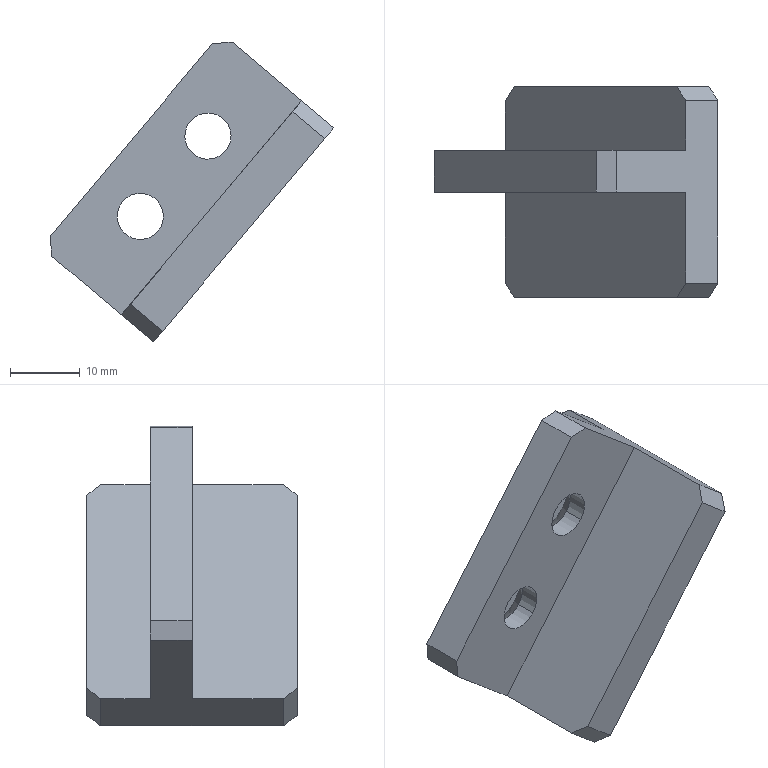Component | SolidWorks | 05CameraLensMountPlate-1 | 1 solid | 24 faces | box 40.54 x 30.1 x 42.84 mm | volume 10080 mm3 | plane 16 | cone 4 | cylinder 4 | commonest cylinder face diameters 6.6 x4 | material Aviation Aluminum-7075
build123d program:
from build123d import *

# Parameters (mm, degrees)
SKETCH1_W                                          = 40
SKETCH1_H                                          = 30.1
BOSS_EXTRUDE1_DEPTH                                = 6
SKETCH2_W                                          = 40
SKETCH2_H                                          = 6
BOSS_EXTRUDE2_DEPTH                                = 15
CHAMFER1_SIZE                                      = 2
HOLE_SIZE_ACCORDING_TO_TYPE_1_OF_HEXAG_D           = 6.6
HOLE_SIZE_ACCORDING_TO_TYPE_1_OF_HEXAG_DEPTH       = 15
HOLE_SIZE_ACCORDING_TO_TYPE_1_OF_HEXAG_CSINK_D     = 12.8
HOLE_SIZE_ACCORDING_TO_TYPE_1_OF_HEXAG_CSINK_ANGLE = 90
HOLE_SIZE_ACCORDING_TO_TYPE_1_OF_HEXAG_TIP         = 1.983


with BuildPart() as part:
    # Sketch1 → Boss-Extrude1 (new body)
    with BuildSketch(Plane.XY):
        Rectangle(SKETCH1_W, SKETCH1_H)
    extrude(amount=BOSS_EXTRUDE1_DEPTH)

    # Sketch2 → Boss-Extrude2 (add)
    with BuildSketch(Plane.XY.offset(6)):
        with Locations((0, -2.95)):
            Rectangle(SKETCH2_W, SKETCH2_H)
    extrude(amount=BOSS_EXTRUDE2_DEPTH)

    # Chamfer1
    chamfer1_edges = [part.edges().sort_by_distance(p)[0] for p in [
        (-20, -2.95, 21),
        (20, -2.95, 21),
        (-20, 15.05, 3),
        (20, 15.05, 3),
        (20, -15.05, 3),
        (-20, -15.05, 3),
    ]]
    chamfer(chamfer1_edges, length=CHAMFER1_SIZE)

    # Hole Size _According to_ Type 1 of Hexag
    with Locations(Plane(origin=(7.5, -5.95, 13), x_dir=(0, 0, -1), z_dir=(0, -1, 0))):
        with Locations((0, 0), (0, -15)):
            CounterSinkHole(HOLE_SIZE_ACCORDING_TO_TYPE_1_OF_HEXAG_D / 2, HOLE_SIZE_ACCORDING_TO_TYPE_1_OF_HEXAG_CSINK_D / 2, depth=HOLE_SIZE_ACCORDING_TO_TYPE_1_OF_HEXAG_DEPTH, counter_sink_angle=HOLE_SIZE_ACCORDING_TO_TYPE_1_OF_HEXAG_CSINK_ANGLE)
            with Locations((0, 0, -(HOLE_SIZE_ACCORDING_TO_TYPE_1_OF_HEXAG_DEPTH + HOLE_SIZE_ACCORDING_TO_TYPE_1_OF_HEXAG_TIP / 2))):  # 118° drill point
                Cone(0, HOLE_SIZE_ACCORDING_TO_TYPE_1_OF_HEXAG_D / 2, HOLE_SIZE_ACCORDING_TO_TYPE_1_OF_HEXAG_TIP, mode=Mode.SUBTRACT)


solid = part.part

# Placed as in the assembly
solid = solid.moved(Location((-338.792, 164.695, -100.519), (0, -49.905, -180)))
STEP:
#1=COLOUR_RGB('',0.7922,0.8196,0.9333);
#2=FILL_AREA_STYLE_COLOUR('',#1);
#3=FILL_AREA_STYLE('',(#2));
#4=SURFACE_STYLE_FILL_AREA(#3);
#5=SURFACE_SIDE_STYLE('',(#4));
#6=SURFACE_STYLE_USAGE(.BOTH.,#5);
#7=PRESENTATION_STYLE_ASSIGNMENT((#6));
#8=CARTESIAN_POINT('',(-14.019,6.596,-3.77));
#9=VERTEX_POINT('',#8);
#10=CARTESIAN_POINT('',(-13.821,6.596,-3.937));
#11=VERTEX_POINT('',#10);
#12=CARTESIAN_POINT('',(-13.92,6.596,-3.854));
#13=DIRECTION('',(-0.,1.,0.));
#14=DIRECTION('',(0.765,0.,-0.6441));
#15=AXIS2_PLACEMENT_3D('',#12,#13,#14);
#16=CIRCLE('',#15,0.1299);
#17=EDGE_CURVE('',#9,#11,#16,.T.);
#18=ORIENTED_EDGE('',*,*,#17,.F.);
#19=CARTESIAN_POINT('',(-14.113,6.718,-3.691));
#20=VERTEX_POINT('',#19);
#21=CARTESIAN_POINT('',(-14.113,6.718,-3.691));
#22=DIRECTION('',(-0.5409,0.7071,0.4554));
#23=VECTOR('',#22,39.37);
#24=LINE('',#21,#23);
#25=EDGE_CURVE('',#9,#20,#24,.T.);
#26=ORIENTED_EDGE('',*,*,#25,.T.);
#27=CARTESIAN_POINT('',(-13.727,6.718,-4.016));
#28=VERTEX_POINT('',#27);
#29=CARTESIAN_POINT('',(-13.92,6.718,-3.854));
#30=DIRECTION('',(-0.,1.,0.));
#31=DIRECTION('',(0.765,0.,-0.6441));
#32=AXIS2_PLACEMENT_3D('',#29,#30,#31);
#33=CIRCLE('',#32,0.252);
#34=EDGE_CURVE('',#20,#28,#33,.T.);
#35=ORIENTED_EDGE('',*,*,#34,.T.);
#36=CARTESIAN_POINT('',(-13.727,6.718,-4.016));
#37=DIRECTION('',(0.5409,0.7071,-0.4554));
#38=VECTOR('',#37,39.37);
#39=LINE('',#36,#38);
#40=EDGE_CURVE('',#11,#28,#39,.T.);
#41=ORIENTED_EDGE('',*,*,#40,.F.);
#42=EDGE_LOOP('',(#18,#26,#35,#41));
#43=FACE_OUTER_BOUND('',#42,.T.);
#44=CARTESIAN_POINT('',(-13.92,6.718,-3.854));
#45=DIRECTION('',(-0.,1.,0.));
#46=DIRECTION('',(0.765,0.,-0.6441));
#47=AXIS2_PLACEMENT_3D('',#44,#45,#46);
#48=CONICAL_SURFACE('',#47,0.252,0.7854);
#49=ADVANCED_FACE('',(#43),#48,.F.);
#50=CARTESIAN_POINT('',(-14.019,6.482,-3.77));
#51=VERTEX_POINT('',#50);
#52=CARTESIAN_POINT('',(-13.821,6.482,-3.937));
#53=VERTEX_POINT('',#52);
#54=CARTESIAN_POINT('',(-13.92,6.482,-3.854));
#55=DIRECTION('',(-0.,1.,0.));
#56=DIRECTION('',(-0.6441,0.,-0.765));
#57=AXIS2_PLACEMENT_3D('',#54,#55,#56);
#58=CIRCLE('',#57,0.1299);
#59=EDGE_CURVE('',#51,#53,#58,.T.);
#60=ORIENTED_EDGE('',*,*,#59,.F.);
#61=CARTESIAN_POINT('',(-14.019,6.718,-3.77));
#62=DIRECTION('',(-0.,1.,0.));
#63=VECTOR('',#62,39.37);
#64=LINE('',#61,#63);
#65=EDGE_CURVE('',#51,#9,#64,.T.);
#66=ORIENTED_EDGE('',*,*,#65,.T.);
#67=ORIENTED_EDGE('',*,*,#17,.T.);
#68=CARTESIAN_POINT('',(-13.821,6.718,-3.937));
#69=DIRECTION('',(-0.,1.,0.));
#70=VECTOR('',#69,39.37);
#71=LINE('',#68,#70);
#72=EDGE_CURVE('',#53,#11,#71,.T.);
#73=ORIENTED_EDGE('',*,*,#72,.F.);
#74=EDGE_LOOP('',(#60,#66,#67,#73));
#75=FACE_OUTER_BOUND('',#74,.T.);
#76=CARTESIAN_POINT('',(-13.92,6.718,-3.854));
#77=DIRECTION('',(-0.,1.,0.));
#78=DIRECTION('',(0.765,0.,-0.6441));
#79=AXIS2_PLACEMENT_3D('',#76,#77,#78);
#80=CYLINDRICAL_SURFACE('',#79,0.1299);
#81=ADVANCED_FACE('',(#75),#80,.F.);
#82=CARTESIAN_POINT('',(-13.639,6.596,-3.318));
#83=VERTEX_POINT('',#82);
#84=CARTESIAN_POINT('',(-13.44,6.596,-3.486));
#85=VERTEX_POINT('',#84);
#86=CARTESIAN_POINT('',(-13.54,6.596,-3.402));
#87=DIRECTION('',(-0.,1.,0.));
#88=DIRECTION('',(0.765,0.,-0.6441));
#89=AXIS2_PLACEMENT_3D('',#86,#87,#88);
#90=CIRCLE('',#89,0.1299);
#91=EDGE_CURVE('',#83,#85,#90,.T.);
#92=ORIENTED_EDGE('',*,*,#91,.F.);
#93=CARTESIAN_POINT('',(-13.732,6.718,-3.24));
#94=VERTEX_POINT('',#93);
#95=CARTESIAN_POINT('',(-13.732,6.718,-3.24));
#96=DIRECTION('',(-0.5409,0.7071,0.4554));
#97=VECTOR('',#96,39.37);
#98=LINE('',#95,#97);
#99=EDGE_CURVE('',#83,#94,#98,.T.);
#100=ORIENTED_EDGE('',*,*,#99,.T.);
#101=CARTESIAN_POINT('',(-13.347,6.718,-3.564));
#102=VERTEX_POINT('',#101);
#103=CARTESIAN_POINT('',(-13.54,6.718,-3.402));
#104=DIRECTION('',(-0.,1.,0.));
#105=DIRECTION('',(0.765,0.,-0.6441));
#106=AXIS2_PLACEMENT_3D('',#103,#104,#105);
#107=CIRCLE('',#106,0.252);
#108=EDGE_CURVE('',#94,#102,#107,.T.);
#109=ORIENTED_EDGE('',*,*,#108,.T.);
#110=CARTESIAN_POINT('',(-13.347,6.718,-3.564));
#111=DIRECTION('',(0.5409,0.7071,-0.4554));
#112=VECTOR('',#111,39.37);
#113=LINE('',#110,#112);
#114=EDGE_CURVE('',#85,#102,#113,.T.);
#115=ORIENTED_EDGE('',*,*,#114,.F.);
#116=EDGE_LOOP('',(#92,#100,#109,#115));
#117=FACE_OUTER_BOUND('',#116,.T.);
#118=CARTESIAN_POINT('',(-13.54,6.718,-3.402));
#119=DIRECTION('',(-0.,1.,0.));
#120=DIRECTION('',(0.765,0.,-0.6441));
#121=AXIS2_PLACEMENT_3D('',#118,#119,#120);
#122=CONICAL_SURFACE('',#121,0.252,0.7854);
#123=ADVANCED_FACE('',(#117),#122,.F.);
#124=CARTESIAN_POINT('',(-13.639,6.482,-3.318));
#125=VERTEX_POINT('',#124);
#126=CARTESIAN_POINT('',(-13.44,6.482,-3.486));
#127=VERTEX_POINT('',#126);
#128=CARTESIAN_POINT('',(-13.54,6.482,-3.402));
#129=DIRECTION('',(-0.,1.,0.));
#130=DIRECTION('',(-0.6441,0.,-0.765));
#131=AXIS2_PLACEMENT_3D('',#128,#129,#130);
#132=CIRCLE('',#131,0.1299);
#133=EDGE_CURVE('',#125,#127,#132,.T.);
#134=ORIENTED_EDGE('',*,*,#133,.F.);
#135=CARTESIAN_POINT('',(-13.639,6.718,-3.318));
#136=DIRECTION('',(-0.,1.,0.));
#137=VECTOR('',#136,39.37);
#138=LINE('',#135,#137);
#139=EDGE_CURVE('',#125,#83,#138,.T.);
#140=ORIENTED_EDGE('',*,*,#139,.T.);
#141=ORIENTED_EDGE('',*,*,#91,.T.);
#142=CARTESIAN_POINT('',(-13.44,6.718,-3.486));
#143=DIRECTION('',(-0.,1.,0.));
#144=VECTOR('',#143,39.37);
#145=LINE('',#142,#144);
#146=EDGE_CURVE('',#127,#85,#145,.T.);
#147=ORIENTED_EDGE('',*,*,#146,.F.);
#148=EDGE_LOOP('',(#134,#140,#141,#147));
#149=FACE_OUTER_BOUND('',#148,.T.);
#150=CARTESIAN_POINT('',(-13.54,6.718,-3.402));
#151=DIRECTION('',(-0.,1.,0.));
#152=DIRECTION('',(0.765,0.,-0.6441));
#153=AXIS2_PLACEMENT_3D('',#150,#151,#152);
#154=CYLINDRICAL_SURFACE('',#153,0.1299);
#155=ADVANCED_FACE('',(#149),#154,.F.);
#156=CARTESIAN_POINT('',(-14.026,6.482,-4.408));
#157=VERTEX_POINT('',#156);
#158=CARTESIAN_POINT('',(-14.026,5.97,-4.408));
#159=VERTEX_POINT('',#158);
#160=CARTESIAN_POINT('',(-14.026,7.077,-4.408));
#161=DIRECTION('',(0.,-1.,-0.));
#162=VECTOR('',#161,39.37);
#163=LINE('',#160,#162);
#164=EDGE_CURVE('',#157,#159,#163,.T.);
#165=ORIENTED_EDGE('',*,*,#164,.T.);
#166=CARTESIAN_POINT('',(-13.975,5.892,-4.347));
#167=VERTEX_POINT('',#166);
#168=CARTESIAN_POINT('',(-13.938,5.833,-4.303));
#169=DIRECTION('',(0.4554,-0.7071,0.5409));
#170=VECTOR('',#169,39.37);
#171=LINE('',#168,#170);
#172=EDGE_CURVE('',#159,#167,#171,.T.);
#173=ORIENTED_EDGE('',*,*,#172,.T.);
#174=CARTESIAN_POINT('',(-13.063,5.892,-3.263));
#175=VERTEX_POINT('',#174);
#176=CARTESIAN_POINT('',(-14.026,5.892,-4.408));
#177=DIRECTION('',(0.6441,0.,0.765));
#178=VECTOR('',#177,39.37);
#179=LINE('',#176,#178);
#180=EDGE_CURVE('',#167,#175,#179,.T.);
#181=ORIENTED_EDGE('',*,*,#180,.T.);
#182=CARTESIAN_POINT('',(-13.012,5.97,-3.203));
#183=VERTEX_POINT('',#182);
#184=CARTESIAN_POINT('',(-13.1,5.833,-3.308));
#185=DIRECTION('',(0.4554,0.7071,0.5409));
#186=VECTOR('',#185,39.37);
#187=LINE('',#184,#186);
#188=EDGE_CURVE('',#175,#183,#187,.T.);
#189=ORIENTED_EDGE('',*,*,#188,.T.);
#190=CARTESIAN_POINT('',(-13.012,6.482,-3.203));
#191=VERTEX_POINT('',#190);
#192=CARTESIAN_POINT('',(-13.012,7.077,-3.203));
#193=DIRECTION('',(-0.,1.,-0.));
#194=VECTOR('',#193,39.37);
#195=LINE('',#192,#194);
#196=EDGE_CURVE('',#183,#191,#195,.T.);
#197=ORIENTED_EDGE('',*,*,#196,.T.);
#198=CARTESIAN_POINT('',(-14.026,6.482,-4.408));
#199=DIRECTION('',(0.6441,0.,0.765));
#200=VECTOR('',#199,39.37);
#201=LINE('',#198,#200);
#202=EDGE_CURVE('',#157,#191,#201,.T.);
#203=ORIENTED_EDGE('',*,*,#202,.F.);
#204=EDGE_LOOP('',(#165,#173,#181,#189,#197,#203));
#205=FACE_OUTER_BOUND('',#204,.T.);
#206=CARTESIAN_POINT('',(-13.519,6.484,-3.805));
#207=DIRECTION('',(-0.765,-0.,0.6441));
#208=DIRECTION('',(-0.6441,-0.,-0.765));
#209=AXIS2_PLACEMENT_3D('',#206,#207,#208);
#210=PLANE('',#209);
#211=ADVANCED_FACE('',(#205),#210,.T.);
#212=CARTESIAN_POINT('',(-13.403,6.718,-2.873));
#213=VERTEX_POINT('',#212);
#214=CARTESIAN_POINT('',(-13.012,6.718,-3.203));
#215=VERTEX_POINT('',#214);
#216=CARTESIAN_POINT('',(-13.464,6.718,-2.823));
#217=DIRECTION('',(0.765,0.,-0.6441));
#218=VECTOR('',#217,39.37);
#219=LINE('',#216,#218);
#220=EDGE_CURVE('',#213,#215,#219,.T.);
#221=ORIENTED_EDGE('',*,*,#220,.F.);
#222=CARTESIAN_POINT('',(-13.403,6.482,-2.873));
#223=VERTEX_POINT('',#222);
#224=CARTESIAN_POINT('',(-13.403,6.482,-2.873));
#225=DIRECTION('',(0.,-1.,0.));
#226=VECTOR('',#225,39.37);
#227=LINE('',#224,#226);
#228=EDGE_CURVE('',#213,#223,#227,.T.);
#229=ORIENTED_EDGE('',*,*,#228,.T.);
#230=CARTESIAN_POINT('',(-13.464,6.482,-2.823));
#231=DIRECTION('',(0.765,0.,-0.6441));
#232=VECTOR('',#231,39.37);
#233=LINE('',#230,#232);
#234=EDGE_CURVE('',#223,#191,#233,.T.);
#235=ORIENTED_EDGE('',*,*,#234,.T.);
#236=ORIENTED_EDGE('',*,*,#196,.F.);
#237=CARTESIAN_POINT('',(-12.831,5.97,-3.355));
#238=VERTEX_POINT('',#237);
#239=CARTESIAN_POINT('',(-13.012,5.97,-3.203));
#240=DIRECTION('',(0.765,0.,-0.6441));
#241=VECTOR('',#240,39.37);
#242=LINE('',#239,#241);
#243=EDGE_CURVE('',#183,#238,#242,.T.);
#244=ORIENTED_EDGE('',*,*,#243,.T.);
#245=CARTESIAN_POINT('',(-12.831,6.998,-3.355));
#246=VERTEX_POINT('',#245);
#247=CARTESIAN_POINT('',(-12.831,7.077,-3.355));
#248=DIRECTION('',(-0.,1.,-0.));
#249=VECTOR('',#248,39.37);
#250=LINE('',#247,#249);
#251=EDGE_CURVE('',#238,#246,#250,.T.);
#252=ORIENTED_EDGE('',*,*,#251,.T.);
#253=CARTESIAN_POINT('',(-13.012,6.998,-3.203));
#254=VERTEX_POINT('',#253);
#255=CARTESIAN_POINT('',(-13.012,6.998,-3.203));
#256=DIRECTION('',(-0.765,-0.,0.6441));
#257=VECTOR('',#256,39.37);
#258=LINE('',#255,#257);
#259=EDGE_CURVE('',#246,#254,#258,.T.);
#260=ORIENTED_EDGE('',*,*,#259,.T.);
#261=CARTESIAN_POINT('',(-13.012,7.077,-3.203));
#262=DIRECTION('',(-0.,1.,-0.));
#263=VECTOR('',#262,39.37);
#264=LINE('',#261,#263);
#265=EDGE_CURVE('',#215,#254,#264,.T.);
#266=ORIENTED_EDGE('',*,*,#265,.F.);
#267=EDGE_LOOP('',(#221,#229,#235,#236,#244,#252,#260,#266));
#268=FACE_OUTER_BOUND('',#267,.T.);
#269=CARTESIAN_POINT('',(-13.012,7.077,-3.203));
#270=DIRECTION('',(-0.6441,-0.,-0.765));
#271=DIRECTION('',(0.,-1.,0.));
#272=AXIS2_PLACEMENT_3D('',#269,#270,#271);
#273=PLANE('',#272);
#274=ADVANCED_FACE('',(#268),#273,.F.);
#275=CARTESIAN_POINT('',(-12.882,7.077,-3.415));
#276=VERTEX_POINT('',#275);
#277=CARTESIAN_POINT('',(-13.795,7.077,-4.5));
#278=VERTEX_POINT('',#277);
#279=CARTESIAN_POINT('',(-13.845,7.077,-4.56));
#280=DIRECTION('',(-0.6441,-0.,-0.765));
#281=VECTOR('',#280,39.37);
#282=LINE('',#279,#281);
#283=EDGE_CURVE('',#276,#278,#282,.T.);
#284=ORIENTED_EDGE('',*,*,#283,.T.);
#285=CARTESIAN_POINT('',(-13.975,7.077,-4.347));
#286=VERTEX_POINT('',#285);
#287=CARTESIAN_POINT('',(-13.975,7.077,-4.347));
#288=DIRECTION('',(-0.765,-0.,0.6441));
#289=VECTOR('',#288,39.37);
#290=LINE('',#287,#289);
#291=EDGE_CURVE('',#278,#286,#290,.T.);
#292=ORIENTED_EDGE('',*,*,#291,.T.);
#293=CARTESIAN_POINT('',(-13.063,7.077,-3.263));
#294=VERTEX_POINT('',#293);
#295=CARTESIAN_POINT('',(-14.026,7.077,-4.408));
#296=DIRECTION('',(-0.6441,-0.,-0.765));
#297=VECTOR('',#296,39.37);
#298=LINE('',#295,#297);
#299=EDGE_CURVE('',#294,#286,#298,.T.);
#300=ORIENTED_EDGE('',*,*,#299,.F.);
#301=CARTESIAN_POINT('',(-13.063,7.077,-3.263));
#302=DIRECTION('',(0.765,0.,-0.6441));
#303=VECTOR('',#302,39.37);
#304=LINE('',#301,#303);
#305=EDGE_CURVE('',#294,#276,#304,.T.);
#306=ORIENTED_EDGE('',*,*,#305,.T.);
#307=EDGE_LOOP('',(#284,#292,#300,#306));
#308=FACE_OUTER_BOUND('',#307,.T.);
#309=CARTESIAN_POINT('',(-14.026,7.077,-4.408));
#310=DIRECTION('',(0.,-1.,0.));
#311=DIRECTION('',(0.6441,0.,0.765));
#312=AXIS2_PLACEMENT_3D('',#309,#310,#311);
#313=PLANE('',#312);
#314=ADVANCED_FACE('',(#308),#313,.F.);
#315=CARTESIAN_POINT('',(-14.418,6.482,-4.078));
#316=VERTEX_POINT('',#315);
#317=CARTESIAN_POINT('',(-14.478,6.482,-4.027));
#318=DIRECTION('',(0.765,0.,-0.6441));
#319=VECTOR('',#318,39.37);
#320=LINE('',#317,#319);
#321=EDGE_CURVE('',#316,#157,#320,.T.);
#322=ORIENTED_EDGE('',*,*,#321,.F.);
#323=CARTESIAN_POINT('',(-14.418,6.718,-4.078));
#324=VERTEX_POINT('',#323);
#325=CARTESIAN_POINT('',(-14.418,6.718,-4.078));
#326=DIRECTION('',(-0.,1.,0.));
#327=VECTOR('',#326,39.37);
#328=LINE('',#325,#327);
#329=EDGE_CURVE('',#316,#324,#328,.T.);
#330=ORIENTED_EDGE('',*,*,#329,.T.);
#331=CARTESIAN_POINT('',(-14.026,6.718,-4.408));
#332=VERTEX_POINT('',#331);
#333=CARTESIAN_POINT('',(-14.478,6.718,-4.027));
#334=DIRECTION('',(0.765,0.,-0.6441));
#335=VECTOR('',#334,39.37);
#336=LINE('',#333,#335);
#337=EDGE_CURVE('',#324,#332,#336,.T.);
#338=ORIENTED_EDGE('',*,*,#337,.T.);
#339=CARTESIAN_POINT('',(-14.026,6.998,-4.408));
#340=VERTEX_POINT('',#339);
#341=CARTESIAN_POINT('',(-14.026,7.077,-4.408));
#342=DIRECTION('',(0.,-1.,-0.));
#343=VECTOR('',#342,39.37);
#344=LINE('',#341,#343);
#345=EDGE_CURVE('',#340,#332,#344,.T.);
#346=ORIENTED_EDGE('',*,*,#345,.F.);
#347=CARTESIAN_POINT('',(-13.845,6.998,-4.56));
#348=VERTEX_POINT('',#347);
#349=CARTESIAN_POINT('',(-14.026,6.998,-4.408));
#350=DIRECTION('',(0.765,0.,-0.6441));
#351=VECTOR('',#350,39.37);
#352=LINE('',#349,#351);
#353=EDGE_CURVE('',#340,#348,#352,.T.);
#354=ORIENTED_EDGE('',*,*,#353,.T.);
#355=CARTESIAN_POINT('',(-13.845,5.97,-4.56));
#356=VERTEX_POINT('',#355);
#357=CARTESIAN_POINT('',(-13.845,7.077,-4.56));
#358=DIRECTION('',(0.,-1.,-0.));
#359=VECTOR('',#358,39.37);
#360=LINE('',#357,#359);
#361=EDGE_CURVE('',#348,#356,#360,.T.);
#362=ORIENTED_EDGE('',*,*,#361,.T.);
#363=CARTESIAN_POINT('',(-14.026,5.97,-4.408));
#364=DIRECTION('',(-0.765,-0.,0.6441));
#365=VECTOR('',#364,39.37);
#366=LINE('',#363,#365);
#367=EDGE_CURVE('',#356,#159,#366,.T.);
#368=ORIENTED_EDGE('',*,*,#367,.T.);
#369=ORIENTED_EDGE('',*,*,#164,.F.);
#370=EDGE_LOOP('',(#322,#330,#338,#346,#354,#362,#368,#369));
#371=FACE_OUTER_BOUND('',#370,.T.);
#372=CARTESIAN_POINT('',(-14.026,7.077,-4.408));
#373=DIRECTION('',(0.6441,0.,0.765));
#374=DIRECTION('',(-0.765,-0.,0.6441));
#375=AXIS2_PLACEMENT_3D('',#372,#373,#374);
#376=PLANE('',#375);
#377=ADVANCED_FACE('',(#371),#376,.F.);
#378=ORIENTED_EDGE('',*,*,#180,.F.);
#379=CARTESIAN_POINT('',(-13.795,5.892,-4.5));
#380=VERTEX_POINT('',#379);
#381=CARTESIAN_POINT('',(-13.975,5.892,-4.347));
#382=DIRECTION('',(0.765,0.,-0.6441));
#383=VECTOR('',#382,39.37);
#384=LINE('',#381,#383);
#385=EDGE_CURVE('',#167,#380,#384,.T.);
#386=ORIENTED_EDGE('',*,*,#385,.T.);
#387=CARTESIAN_POINT('',(-12.882,5.892,-3.415));
#388=VERTEX_POINT('',#387);
#389=CARTESIAN_POINT('',(-13.845,5.892,-4.56));
#390=DIRECTION('',(0.6441,0.,0.765));
#391=VECTOR('',#390,39.37);
#392=LINE('',#389,#391);
#393=EDGE_CURVE('',#380,#388,#392,.T.);
#394=ORIENTED_EDGE('',*,*,#393,.T.);
#395=CARTESIAN_POINT('',(-13.063,5.892,-3.263));
#396=DIRECTION('',(-0.765,-0.,0.6441));
#397=VECTOR('',#396,39.37);
#398=LINE('',#395,#397);
#399=EDGE_CURVE('',#388,#175,#398,.T.);
#400=ORIENTED_EDGE('',*,*,#399,.T.);
#401=EDGE_LOOP('',(#378,#386,#394,#400));
#402=FACE_OUTER_BOUND('',#401,.T.);
#403=CARTESIAN_POINT('',(-14.026,5.892,-4.408));
#404=DIRECTION('',(-0.,1.,-0.));
#405=DIRECTION('',(-0.6441,-0.,-0.765));
#406=AXIS2_PLACEMENT_3D('',#403,#404,#405);
#407=PLANE('',#406);
#408=ADVANCED_FACE('',(#402),#407,.F.);
#409=ORIENTED_EDGE('',*,*,#299,.T.);
#410=CARTESIAN_POINT('',(-13.938,7.135,-4.303));
#411=DIRECTION('',(-0.4554,-0.7071,-0.5409));
#412=VECTOR('',#411,39.37);
#413=LINE('',#410,#412);
#414=EDGE_CURVE('',#286,#340,#413,.T.);
#415=ORIENTED_EDGE('',*,*,#414,.T.);
#416=ORIENTED_EDGE('',*,*,#345,.T.);
#417=CARTESIAN_POINT('',(-14.026,6.718,-4.408));
#418=DIRECTION('',(-0.6441,-0.,-0.765));
#419=VECTOR('',#418,39.37);
#420=LINE('',#417,#419);
#421=EDGE_CURVE('',#215,#332,#420,.T.);
#422=ORIENTED_EDGE('',*,*,#421,.F.);
#423=ORIENTED_EDGE('',*,*,#265,.T.);
#424=CARTESIAN_POINT('',(-13.1,7.135,-3.308));
#425=DIRECTION('',(-0.4554,0.7071,-0.5409));
#426=VECTOR('',#425,39.37);
#427=LINE('',#424,#426);
#428=EDGE_CURVE('',#254,#294,#427,.T.);
#429=ORIENTED_EDGE('',*,*,#428,.T.);
#430=EDGE_LOOP('',(#409,#415,#416,#422,#423,#429));
#431=FACE_OUTER_BOUND('',#430,.T.);
#432=CARTESIAN_POINT('',(-13.519,6.484,-3.805));
#433=DIRECTION('',(-0.765,-0.,0.6441));
#434=DIRECTION('',(-0.6441,-0.,-0.765));
#435=AXIS2_PLACEMENT_3D('',#432,#433,#434);
#436=PLANE('',#435);
#437=ADVANCED_FACE('',(#431),#436,.T.);
#438=ORIENTED_EDGE('',*,*,#393,.F.);
#439=CARTESIAN_POINT('',(-13.795,5.892,-4.5));
#440=DIRECTION('',(-0.4554,0.7071,-0.5409));
#441=VECTOR('',#440,39.37);
#442=LINE('',#439,#441);
#443=EDGE_CURVE('',#380,#356,#442,.T.);
#444=ORIENTED_EDGE('',*,*,#443,.T.);
#445=ORIENTED_EDGE('',*,*,#361,.F.);
#446=CARTESIAN_POINT('',(-13.845,6.998,-4.56));
#447=DIRECTION('',(0.4554,0.7071,0.5409));
#448=VECTOR('',#447,39.37);
#449=LINE('',#446,#448);
#450=EDGE_CURVE('',#348,#278,#449,.T.);
#451=ORIENTED_EDGE('',*,*,#450,.T.);
#452=ORIENTED_EDGE('',*,*,#283,.F.);
#453=CARTESIAN_POINT('',(-12.882,7.077,-3.415));
#454=DIRECTION('',(0.4554,-0.7071,0.5409));
#455=VECTOR('',#454,39.37);
#456=LINE('',#453,#455);
#457=EDGE_CURVE('',#276,#246,#456,.T.);
#458=ORIENTED_EDGE('',*,*,#457,.T.);
#459=ORIENTED_EDGE('',*,*,#251,.F.);
#460=CARTESIAN_POINT('',(-12.831,5.97,-3.355));
#461=DIRECTION('',(-0.4554,-0.7071,-0.5409));
#462=VECTOR('',#461,39.37);
#463=LINE('',#460,#462);
#464=EDGE_CURVE('',#238,#388,#463,.T.);
#465=ORIENTED_EDGE('',*,*,#464,.T.);
#466=EDGE_LOOP('',(#438,#444,#445,#451,#452,#458,#459,#465));
#467=FACE_OUTER_BOUND('',#466,.T.);
#468=CARTESIAN_POINT('',(-13.338,6.484,-3.957));
#469=DIRECTION('',(-0.765,-0.,0.6441));
#470=DIRECTION('',(-0.6441,-0.,-0.765));
#471=AXIS2_PLACEMENT_3D('',#468,#469,#470);
#472=PLANE('',#471);
#473=ADVANCED_FACE('',(#467),#472,.F.);
#474=CARTESIAN_POINT('',(-13.92,6.718,-3.854));
#475=DIRECTION('',(-0.,1.,0.));
#476=DIRECTION('',(0.765,0.,-0.6441));
#477=AXIS2_PLACEMENT_3D('',#474,#475,#476);
#478=CIRCLE('',#477,0.252);
#479=EDGE_CURVE('',#28,#20,#478,.T.);
#480=ORIENTED_EDGE('',*,*,#479,.F.);
#481=ORIENTED_EDGE('',*,*,#34,.F.);
#482=EDGE_LOOP('',(#480,#481));
#483=FACE_BOUND('',#482,.T.);
#484=CARTESIAN_POINT('',(-13.54,6.718,-3.402));
#485=DIRECTION('',(-0.,1.,0.));
#486=DIRECTION('',(0.765,0.,-0.6441));
#487=AXIS2_PLACEMENT_3D('',#484,#485,#486);
#488=CIRCLE('',#487,0.252);
#489=EDGE_CURVE('',#102,#94,#488,.T.);
#490=ORIENTED_EDGE('',*,*,#489,.F.);
#491=ORIENTED_EDGE('',*,*,#108,.F.);
#492=EDGE_LOOP('',(#490,#491));
#493=FACE_BOUND('',#492,.T.);
#494=ORIENTED_EDGE('',*,*,#337,.F.);
#495=CARTESIAN_POINT('',(-14.427,6.718,-3.967));
#496=VERTEX_POINT('',#495);
#497=CARTESIAN_POINT('',(-14.427,6.718,-3.967));
#498=DIRECTION('',(-0.0855,-0.,0.9963));
#499=VECTOR('',#498,39.37);
#500=LINE('',#497,#499);
#501=EDGE_CURVE('',#324,#496,#500,.T.);
#502=ORIENTED_EDGE('',*,*,#501,.T.);
#503=CARTESIAN_POINT('',(-13.514,6.718,-2.883));
#504=VERTEX_POINT('',#503);
#505=CARTESIAN_POINT('',(-14.478,6.718,-4.027));
#506=DIRECTION('',(-0.6441,-0.,-0.765));
#507=VECTOR('',#506,39.37);
#508=LINE('',#505,#507);
#509=EDGE_CURVE('',#504,#496,#508,.T.);
#510=ORIENTED_EDGE('',*,*,#509,.F.);
#511=CARTESIAN_POINT('',(-13.514,6.718,-2.883));
#512=DIRECTION('',(0.9963,0.,0.0855));
#513=VECTOR('',#512,39.37);
#514=LINE('',#511,#513);
#515=EDGE_CURVE('',#504,#213,#514,.T.);
#516=ORIENTED_EDGE('',*,*,#515,.T.);
#517=ORIENTED_EDGE('',*,*,#220,.T.);
#518=ORIENTED_EDGE('',*,*,#421,.T.);
#519=EDGE_LOOP('',(#494,#502,#510,#516,#517,#518));
#520=FACE_OUTER_BOUND('',#519,.T.);
#521=CARTESIAN_POINT('',(-14.478,6.718,-4.027));
#522=DIRECTION('',(0.,-1.,-0.));
#523=DIRECTION('',(-0.765,-0.,0.6441));
#524=AXIS2_PLACEMENT_3D('',#521,#522,#523);
#525=PLANE('',#524);
#526=ADVANCED_FACE('',(#483,#493,#520),#525,.F.);
#527=CARTESIAN_POINT('',(-13.92,6.482,-3.854));
#528=DIRECTION('',(-0.,1.,0.));
#529=DIRECTION('',(-0.6441,0.,-0.765));
#530=AXIS2_PLACEMENT_3D('',#527,#528,#529);
#531=CIRCLE('',#530,0.1299);
#532=EDGE_CURVE('',#53,#51,#531,.T.);
#533=ORIENTED_EDGE('',*,*,#532,.T.);
#534=ORIENTED_EDGE('',*,*,#59,.T.);
#535=EDGE_LOOP('',(#533,#534));
#536=FACE_BOUND('',#535,.T.);
#537=CARTESIAN_POINT('',(-13.54,6.482,-3.402));
#538=DIRECTION('',(-0.,1.,0.));
#539=DIRECTION('',(-0.6441,0.,-0.765));
#540=AXIS2_PLACEMENT_3D('',#537,#538,#539);
#541=CIRCLE('',#540,0.1299);
#542=EDGE_CURVE('',#127,#125,#541,.T.);
#543=ORIENTED_EDGE('',*,*,#542,.T.);
#544=ORIENTED_EDGE('',*,*,#133,.T.);
#545=EDGE_LOOP('',(#543,#544));
#546=FACE_BOUND('',#545,.T.);
#547=CARTESIAN_POINT('',(-14.427,6.482,-3.967));
#548=VERTEX_POINT('',#547);
#549=CARTESIAN_POINT('',(-13.514,6.482,-2.883));
#550=VERTEX_POINT('',#549);
#551=CARTESIAN_POINT('',(-14.478,6.482,-4.027));
#552=DIRECTION('',(0.6441,0.,0.765));
#553=VECTOR('',#552,39.37);
#554=LINE('',#551,#553);
#555=EDGE_CURVE('',#548,#550,#554,.T.);
#556=ORIENTED_EDGE('',*,*,#555,.F.);
#557=CARTESIAN_POINT('',(-14.427,6.482,-3.967));
#558=DIRECTION('',(0.0855,0.,-0.9963));
#559=VECTOR('',#558,39.37);
#560=LINE('',#557,#559);
#561=EDGE_CURVE('',#548,#316,#560,.T.);
#562=ORIENTED_EDGE('',*,*,#561,.T.);
#563=ORIENTED_EDGE('',*,*,#321,.T.);
#564=ORIENTED_EDGE('',*,*,#202,.T.);
#565=ORIENTED_EDGE('',*,*,#234,.F.);
#566=CARTESIAN_POINT('',(-13.514,6.482,-2.883));
#567=DIRECTION('',(-0.9963,-0.,-0.0855));
#568=VECTOR('',#567,39.37);
#569=LINE('',#566,#568);
#570=EDGE_CURVE('',#223,#550,#569,.T.);
#571=ORIENTED_EDGE('',*,*,#570,.T.);
#572=EDGE_LOOP('',(#556,#562,#563,#564,#565,#571));
#573=FACE_OUTER_BOUND('',#572,.T.);
#574=CARTESIAN_POINT('',(-14.478,6.482,-4.027));
#575=DIRECTION('',(-0.,1.,0.));
#576=DIRECTION('',(-0.6441,-0.,-0.765));
#577=AXIS2_PLACEMENT_3D('',#574,#575,#576);
#578=PLANE('',#577);
#579=ADVANCED_FACE('',(#536,#546,#573),#578,.F.);
#580=ORIENTED_EDGE('',*,*,#509,.T.);
#581=CARTESIAN_POINT('',(-14.427,6.482,-3.967));
#582=DIRECTION('',(0.,-1.,-0.));
#583=VECTOR('',#582,39.37);
#584=LINE('',#581,#583);
#585=EDGE_CURVE('',#496,#548,#584,.T.);
#586=ORIENTED_EDGE('',*,*,#585,.T.);
#587=ORIENTED_EDGE('',*,*,#555,.T.);
#588=CARTESIAN_POINT('',(-13.514,6.718,-2.883));
#589=DIRECTION('',(-0.,1.,-0.));
#590=VECTOR('',#589,39.37);
#591=LINE('',#588,#590);
#592=EDGE_CURVE('',#550,#504,#591,.T.);
#593=ORIENTED_EDGE('',*,*,#592,.T.);
#594=EDGE_LOOP('',(#580,#586,#587,#593));
#595=FACE_OUTER_BOUND('',#594,.T.);
#596=CARTESIAN_POINT('',(-13.971,6.484,-3.425));
#597=DIRECTION('',(-0.765,-0.,0.6441));
#598=DIRECTION('',(-0.6441,-0.,-0.765));
#599=AXIS2_PLACEMENT_3D('',#596,#597,#598);
#600=PLANE('',#599);
#601=ADVANCED_FACE('',(#595),#600,.T.);
#602=ORIENTED_EDGE('',*,*,#501,.F.);
#603=ORIENTED_EDGE('',*,*,#329,.F.);
#604=ORIENTED_EDGE('',*,*,#561,.F.);
#605=ORIENTED_EDGE('',*,*,#585,.F.);
#606=EDGE_LOOP('',(#602,#603,#604,#605));
#607=FACE_OUTER_BOUND('',#606,.T.);
#608=CARTESIAN_POINT('',(-14.427,6.484,-3.967));
#609=DIRECTION('',(-0.9963,-0.,-0.0855));
#610=DIRECTION('',(-0.,1.,0.));
#611=AXIS2_PLACEMENT_3D('',#608,#609,#610);
#612=PLANE('',#611);
#613=ADVANCED_FACE('',(#607),#612,.T.);
#614=ORIENTED_EDGE('',*,*,#570,.F.);
#615=ORIENTED_EDGE('',*,*,#228,.F.);
#616=ORIENTED_EDGE('',*,*,#515,.F.);
#617=ORIENTED_EDGE('',*,*,#592,.F.);
#618=EDGE_LOOP('',(#614,#615,#616,#617));
#619=FACE_OUTER_BOUND('',#618,.T.);
#620=CARTESIAN_POINT('',(-13.514,6.484,-2.883));
#621=DIRECTION('',(-0.0855,0.,0.9963));
#622=DIRECTION('',(0.,-1.,0.));
#623=AXIS2_PLACEMENT_3D('',#620,#621,#622);
#624=PLANE('',#623);
#625=ADVANCED_FACE('',(#619),#624,.T.);
#626=ORIENTED_EDGE('',*,*,#172,.F.);
#627=ORIENTED_EDGE('',*,*,#367,.F.);
#628=ORIENTED_EDGE('',*,*,#443,.F.);
#629=ORIENTED_EDGE('',*,*,#385,.F.);
#630=EDGE_LOOP('',(#626,#627,#628,#629));
#631=FACE_OUTER_BOUND('',#630,.T.);
#632=CARTESIAN_POINT('',(-13.975,5.892,-4.347));
#633=DIRECTION('',(0.4554,0.7071,0.5409));
#634=DIRECTION('',(0.765,0.,-0.6441));
#635=AXIS2_PLACEMENT_3D('',#632,#633,#634);
#636=PLANE('',#635);
#637=ADVANCED_FACE('',(#631),#636,.F.);
#638=ORIENTED_EDGE('',*,*,#188,.F.);
#639=ORIENTED_EDGE('',*,*,#399,.F.);
#640=ORIENTED_EDGE('',*,*,#464,.F.);
#641=ORIENTED_EDGE('',*,*,#243,.F.);
#642=EDGE_LOOP('',(#638,#639,#640,#641));
#643=FACE_OUTER_BOUND('',#642,.T.);
#644=CARTESIAN_POINT('',(-13.012,5.97,-3.203));
#645=DIRECTION('',(-0.4554,0.7071,-0.5409));
#646=DIRECTION('',(0.765,0.,-0.6441));
#647=AXIS2_PLACEMENT_3D('',#644,#645,#646);
#648=PLANE('',#647);
#649=ADVANCED_FACE('',(#643),#648,.F.);
#650=ORIENTED_EDGE('',*,*,#414,.F.);
#651=ORIENTED_EDGE('',*,*,#291,.F.);
#652=ORIENTED_EDGE('',*,*,#450,.F.);
#653=ORIENTED_EDGE('',*,*,#353,.F.);
#654=EDGE_LOOP('',(#650,#651,#652,#653));
#655=FACE_OUTER_BOUND('',#654,.T.);
#656=CARTESIAN_POINT('',(-14.026,6.998,-4.408));
#657=DIRECTION('',(0.4554,-0.7071,0.5409));
#658=DIRECTION('',(0.765,0.,-0.6441));
#659=AXIS2_PLACEMENT_3D('',#656,#657,#658);
#660=PLANE('',#659);
#661=ADVANCED_FACE('',(#655),#660,.F.);
#662=ORIENTED_EDGE('',*,*,#428,.F.);
#663=ORIENTED_EDGE('',*,*,#259,.F.);
#664=ORIENTED_EDGE('',*,*,#457,.F.);
#665=ORIENTED_EDGE('',*,*,#305,.F.);
#666=EDGE_LOOP('',(#662,#663,#664,#665));
#667=FACE_OUTER_BOUND('',#666,.T.);
#668=CARTESIAN_POINT('',(-13.063,7.077,-3.263));
#669=DIRECTION('',(-0.4554,-0.7071,-0.5409));
#670=DIRECTION('',(0.765,0.,-0.6441));
#671=AXIS2_PLACEMENT_3D('',#668,#669,#670);
#672=PLANE('',#671);
#673=ADVANCED_FACE('',(#667),#672,.F.);
#674=ORIENTED_EDGE('',*,*,#139,.F.);
#675=ORIENTED_EDGE('',*,*,#542,.F.);
#676=ORIENTED_EDGE('',*,*,#146,.T.);
#677=CARTESIAN_POINT('',(-13.54,6.596,-3.402));
#678=DIRECTION('',(-0.,1.,0.));
#679=DIRECTION('',(0.765,0.,-0.6441));
#680=AXIS2_PLACEMENT_3D('',#677,#678,#679);
#681=CIRCLE('',#680,0.1299);
#682=EDGE_CURVE('',#85,#83,#681,.T.);
#683=ORIENTED_EDGE('',*,*,#682,.T.);
#684=EDGE_LOOP('',(#674,#675,#676,#683));
#685=FACE_OUTER_BOUND('',#684,.T.);
#686=CARTESIAN_POINT('',(-13.54,6.718,-3.402));
#687=DIRECTION('',(-0.,1.,0.));
#688=DIRECTION('',(0.765,0.,-0.6441));
#689=AXIS2_PLACEMENT_3D('',#686,#687,#688);
#690=CYLINDRICAL_SURFACE('',#689,0.1299);
#691=ADVANCED_FACE('',(#685),#690,.F.);
#692=ORIENTED_EDGE('',*,*,#99,.F.);
#693=ORIENTED_EDGE('',*,*,#682,.F.);
#694=ORIENTED_EDGE('',*,*,#114,.T.);
#695=ORIENTED_EDGE('',*,*,#489,.T.);
#696=EDGE_LOOP('',(#692,#693,#694,#695));
#697=FACE_OUTER_BOUND('',#696,.T.);
#698=CARTESIAN_POINT('',(-13.54,6.718,-3.402));
#699=DIRECTION('',(-0.,1.,0.));
#700=DIRECTION('',(0.765,0.,-0.6441));
#701=AXIS2_PLACEMENT_3D('',#698,#699,#700);
#702=CONICAL_SURFACE('',#701,0.252,0.7854);
#703=ADVANCED_FACE('',(#697),#702,.F.);
#704=ORIENTED_EDGE('',*,*,#65,.F.);
#705=ORIENTED_EDGE('',*,*,#532,.F.);
#706=ORIENTED_EDGE('',*,*,#72,.T.);
#707=CARTESIAN_POINT('',(-13.92,6.596,-3.854));
#708=DIRECTION('',(-0.,1.,0.));
#709=DIRECTION('',(0.765,0.,-0.6441));
#710=AXIS2_PLACEMENT_3D('',#707,#708,#709);
#711=CIRCLE('',#710,0.1299);
#712=EDGE_CURVE('',#11,#9,#711,.T.);
#713=ORIENTED_EDGE('',*,*,#712,.T.);
#714=EDGE_LOOP('',(#704,#705,#706,#713));
#715=FACE_OUTER_BOUND('',#714,.T.);
#716=CARTESIAN_POINT('',(-13.92,6.718,-3.854));
#717=DIRECTION('',(-0.,1.,0.));
#718=DIRECTION('',(0.765,0.,-0.6441));
#719=AXIS2_PLACEMENT_3D('',#716,#717,#718);
#720=CYLINDRICAL_SURFACE('',#719,0.1299);
#721=ADVANCED_FACE('',(#715),#720,.F.);
#722=ORIENTED_EDGE('',*,*,#25,.F.);
#723=ORIENTED_EDGE('',*,*,#712,.F.);
#724=ORIENTED_EDGE('',*,*,#40,.T.);
#725=ORIENTED_EDGE('',*,*,#479,.T.);
#726=EDGE_LOOP('',(#722,#723,#724,#725));
#727=FACE_OUTER_BOUND('',#726,.T.);
#728=CARTESIAN_POINT('',(-13.92,6.718,-3.854));
#729=DIRECTION('',(-0.,1.,0.));
#730=DIRECTION('',(0.765,0.,-0.6441));
#731=AXIS2_PLACEMENT_3D('',#728,#729,#730);
#732=CONICAL_SURFACE('',#731,0.252,0.7854);
#733=ADVANCED_FACE('',(#727),#732,.F.);
#734=CLOSED_SHELL('',(#49,#81,#123,#155,#211,#274,#314,#377,#408,#437,#473,#526,#579,#601,#613,#625,#637,#649,#661,#673,#691,#703,#721,#733));
#735=MANIFOLD_SOLID_BREP('',#734);
#736=STYLED_ITEM('',(#7),#735);
#737=PRESENTATION_LAYER_ASSIGNMENT('','',(#736));
#738=CARTESIAN_POINT('',(0.,0.,0.));
#739=DIRECTION('',(0.,0.,1.));
#740=DIRECTION('',(1.,0.,0.));
#741=AXIS2_PLACEMENT_3D('',#738,#739,#740);
#742=(LENGTH_UNIT()NAMED_UNIT(*)SI_UNIT($,.METRE.));
#743=LENGTH_MEASURE_WITH_UNIT(LENGTH_MEASURE(0.0254),#742);
#744=DIMENSIONAL_EXPONENTS(1.,0.,0.,0.,0.,0.,0.);
#745=(CONVERSION_BASED_UNIT('',#743)LENGTH_UNIT()NAMED_UNIT(#744));
#746=UNCERTAINTY_MEASURE_WITH_UNIT(LENGTH_MEASURE(0.00001),#745,'','');
#747=(NAMED_UNIT(*)PLANE_ANGLE_UNIT()SI_UNIT($,.RADIAN.));
#748=(NAMED_UNIT(*)SI_UNIT($,.STERADIAN.)SOLID_ANGLE_UNIT());
#749=(GEOMETRIC_REPRESENTATION_CONTEXT(3)GLOBAL_UNCERTAINTY_ASSIGNED_CONTEXT((#746))GLOBAL_UNIT_ASSIGNED_CONTEXT((#745,#747,#748))REPRESENTATION_CONTEXT('',''));
#750=ADVANCED_BREP_SHAPE_REPRESENTATION('',(#735,#741),#749);
#751=(LENGTH_UNIT()NAMED_UNIT(*)SI_UNIT($,.METRE.));
#752=LENGTH_MEASURE_WITH_UNIT(LENGTH_MEASURE(0.0254),#751);
#753=DIMENSIONAL_EXPONENTS(1.,0.,0.,0.,0.,0.,0.);
#754=(CONVERSION_BASED_UNIT('',#752)LENGTH_UNIT()NAMED_UNIT(#753));
#755=UNCERTAINTY_MEASURE_WITH_UNIT(LENGTH_MEASURE(0.00001),#754,'','');
#756=(NAMED_UNIT(*)PLANE_ANGLE_UNIT()SI_UNIT($,.RADIAN.));
#757=(NAMED_UNIT(*)SI_UNIT($,.STERADIAN.)SOLID_ANGLE_UNIT());
#758=(GEOMETRIC_REPRESENTATION_CONTEXT(3)GLOBAL_UNCERTAINTY_ASSIGNED_CONTEXT((#755))GLOBAL_UNIT_ASSIGNED_CONTEXT((#754,#756,#757))REPRESENTATION_CONTEXT('',''));
#759=MECHANICAL_DESIGN_GEOMETRIC_PRESENTATION_REPRESENTATION('',(#736),#758);